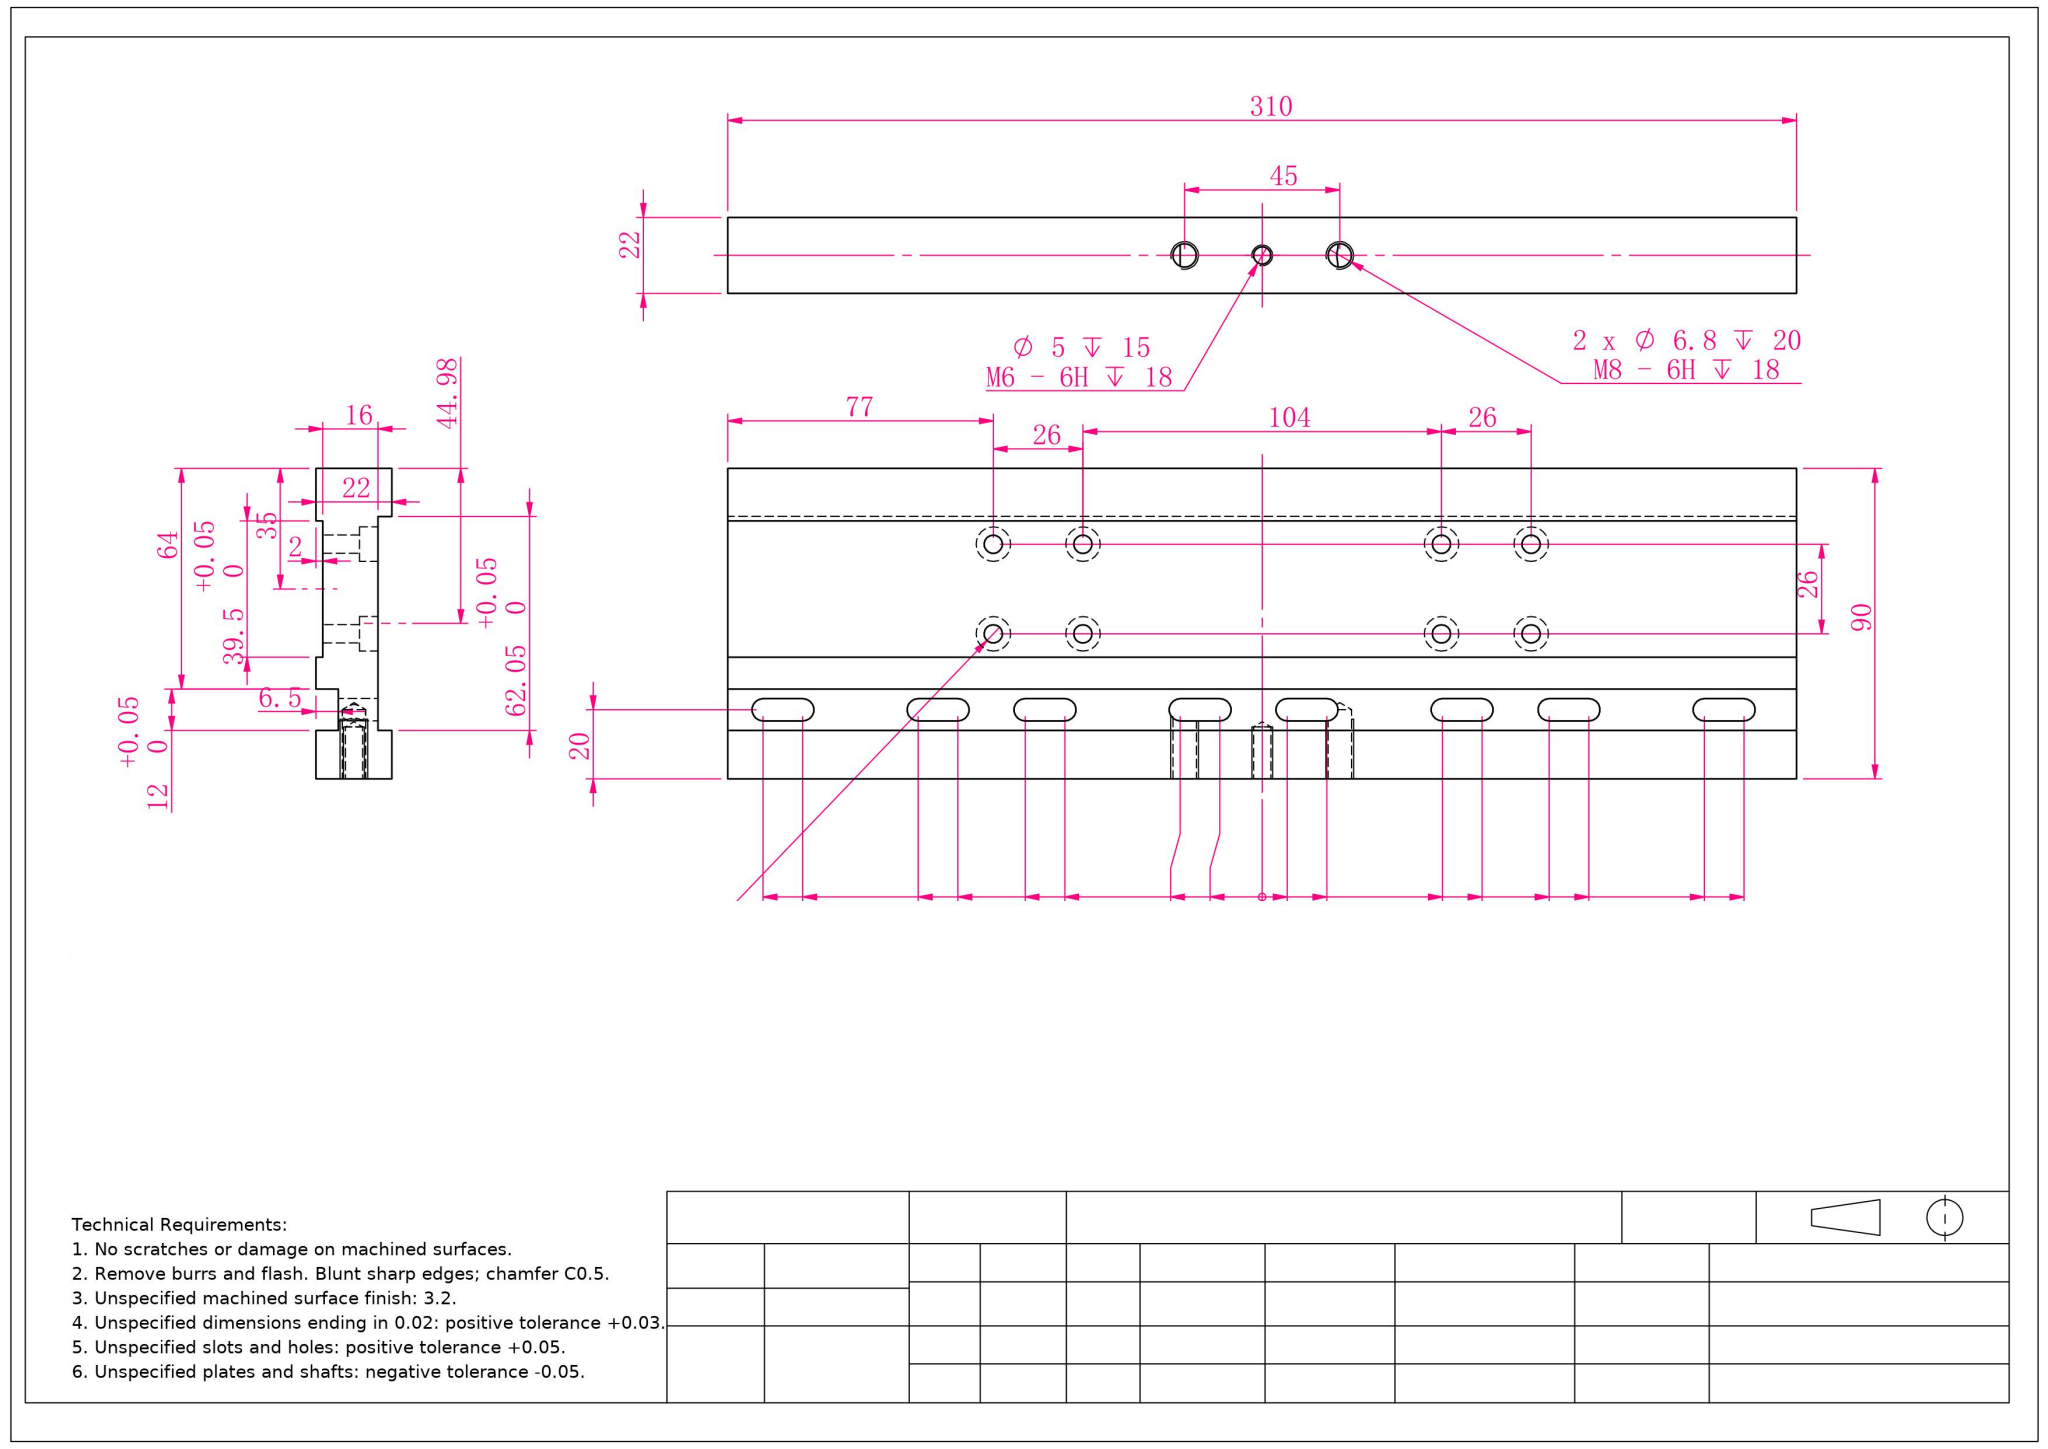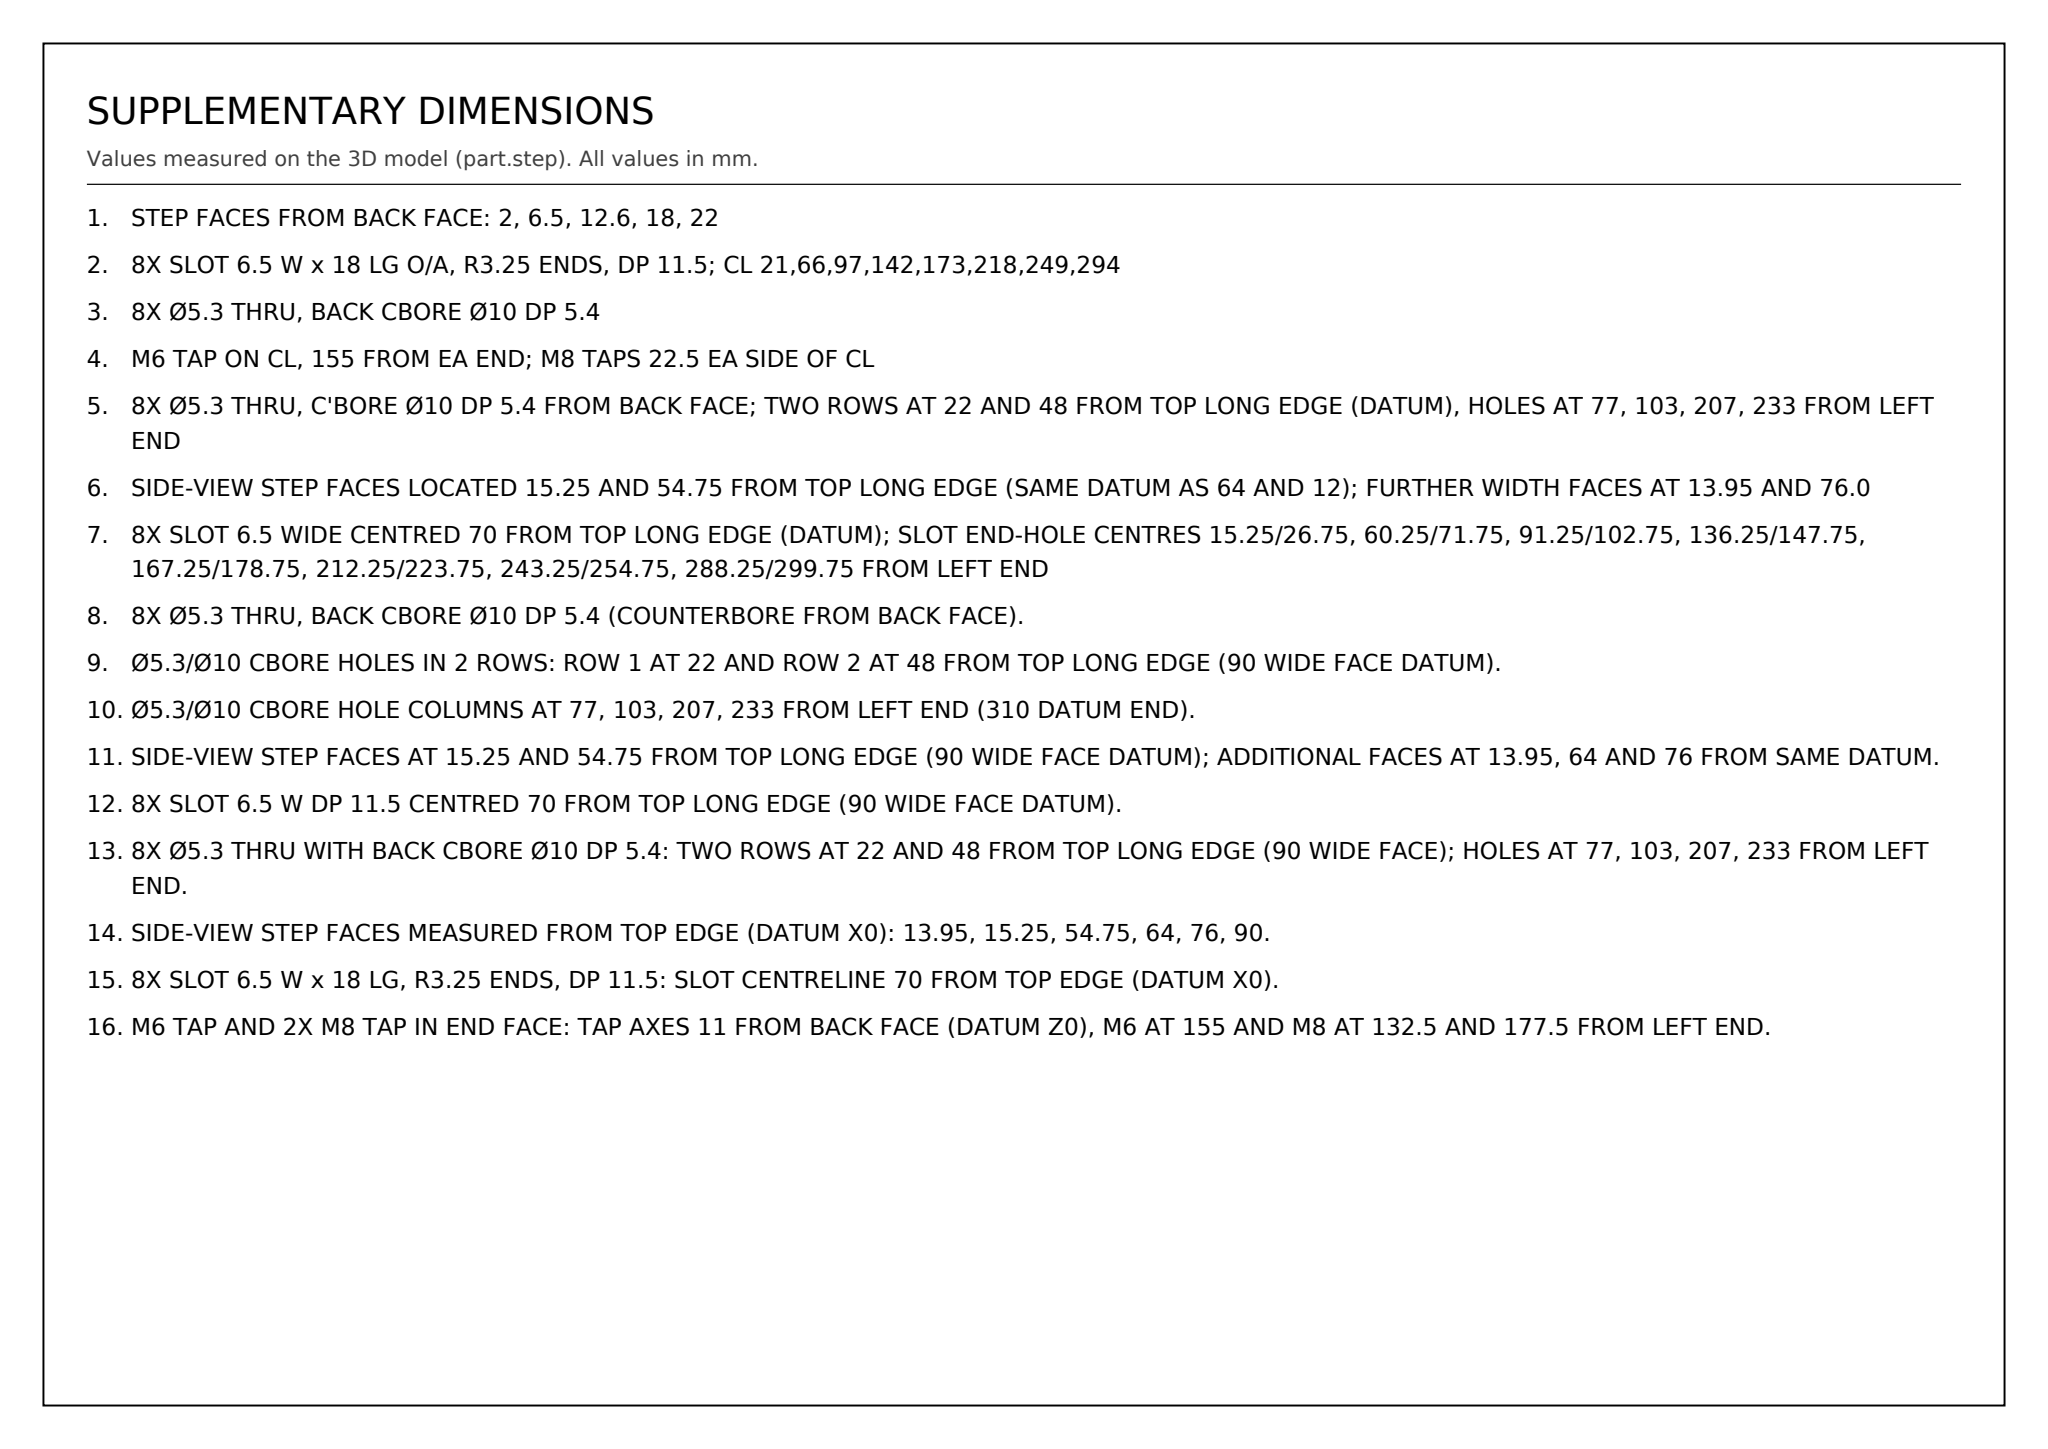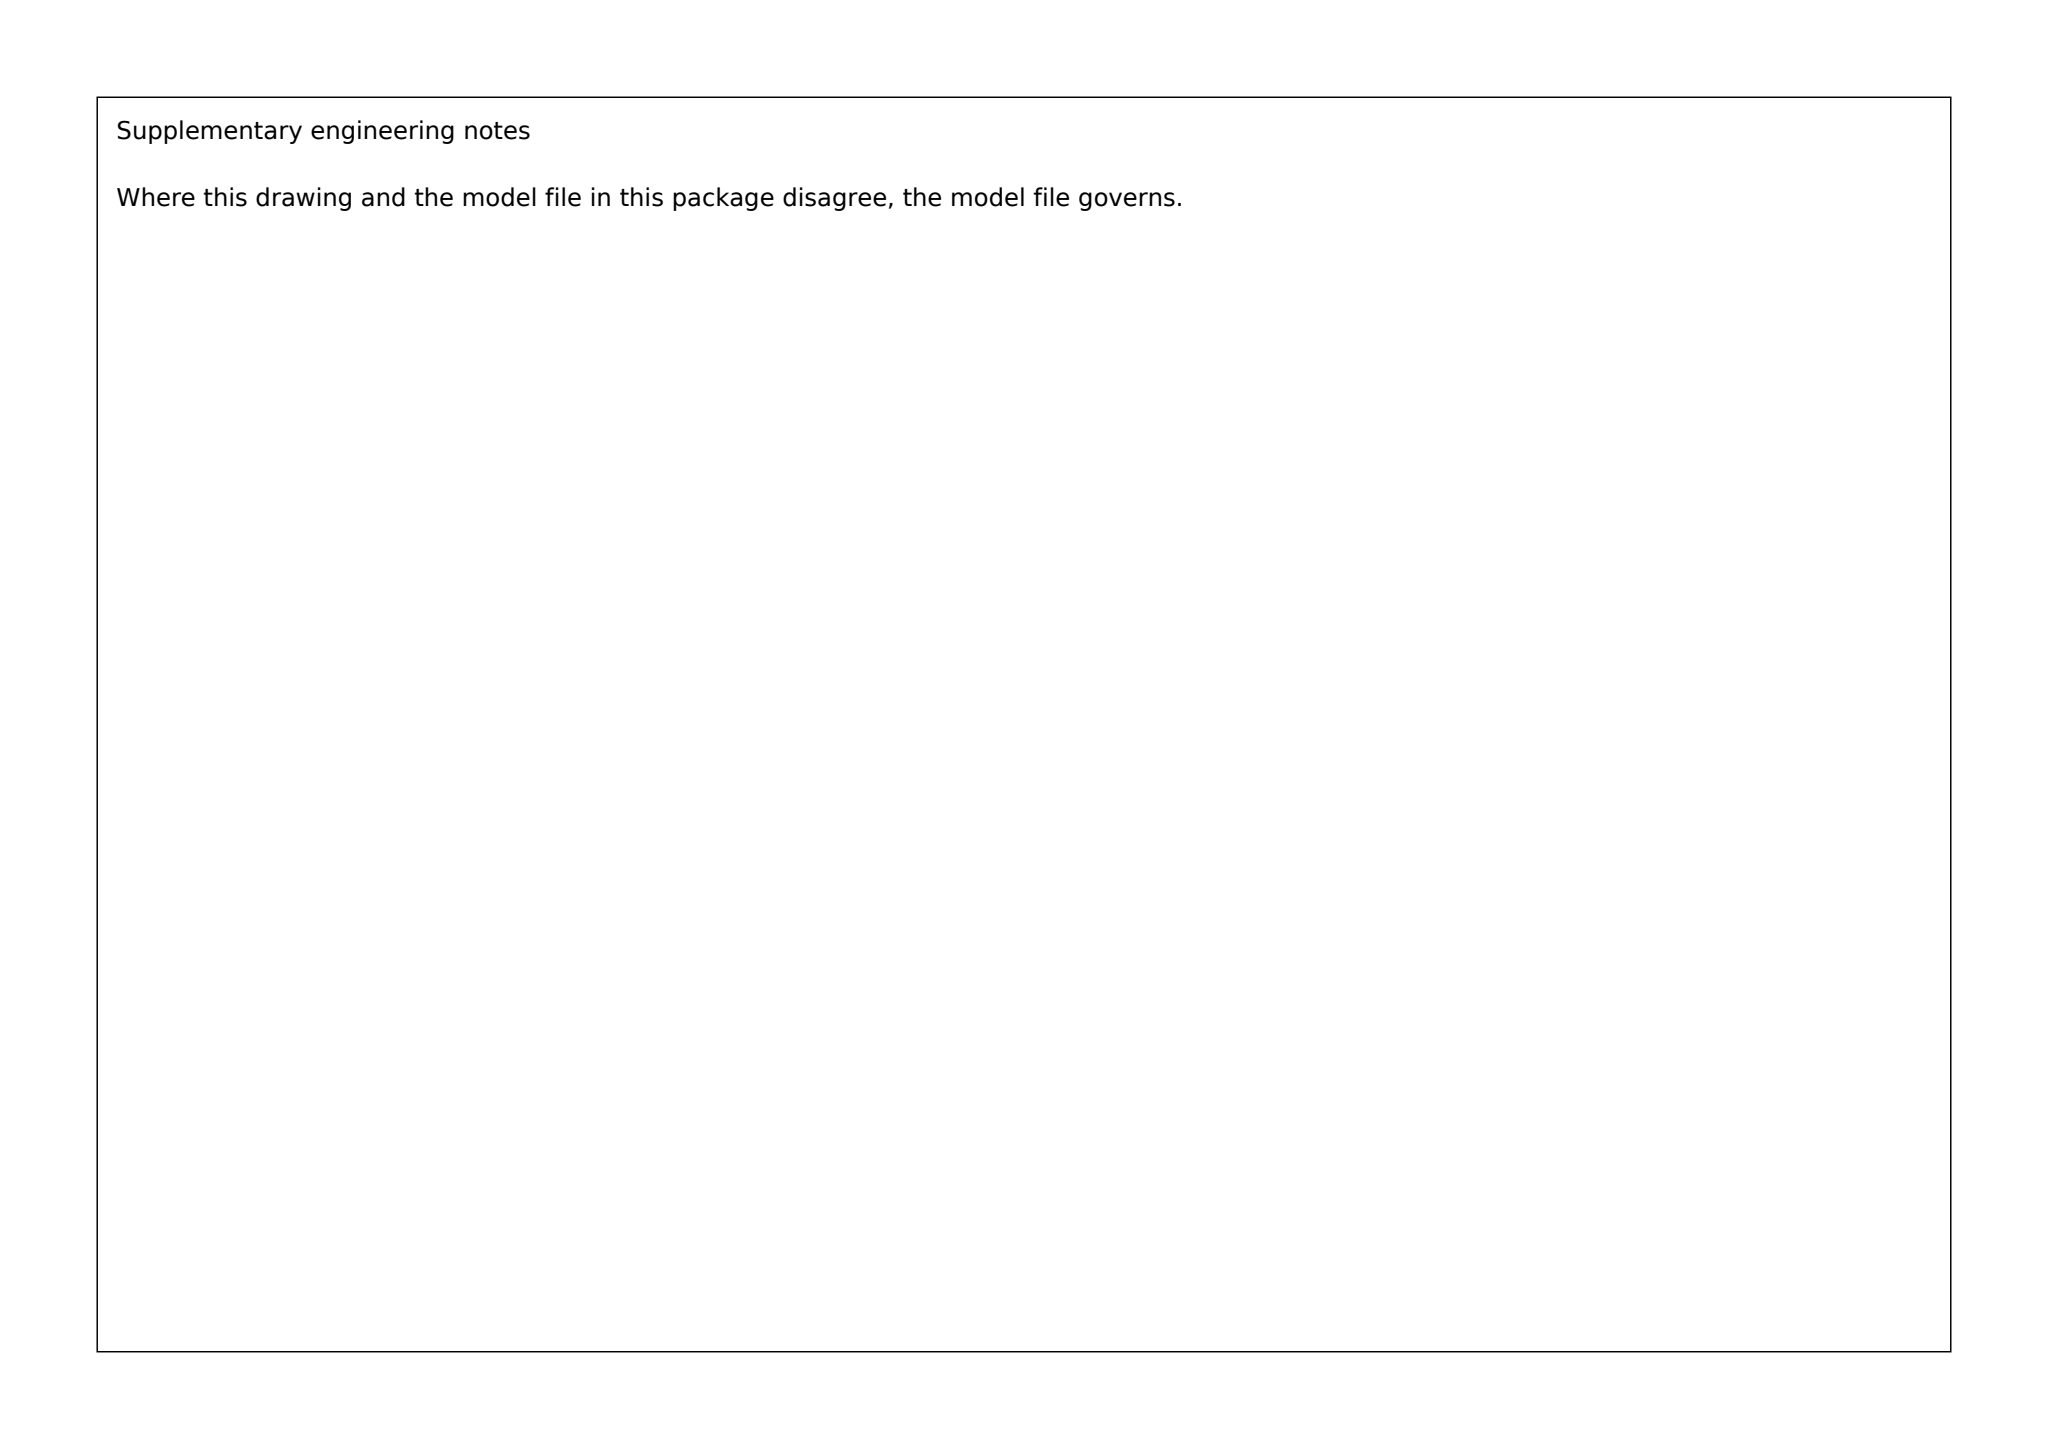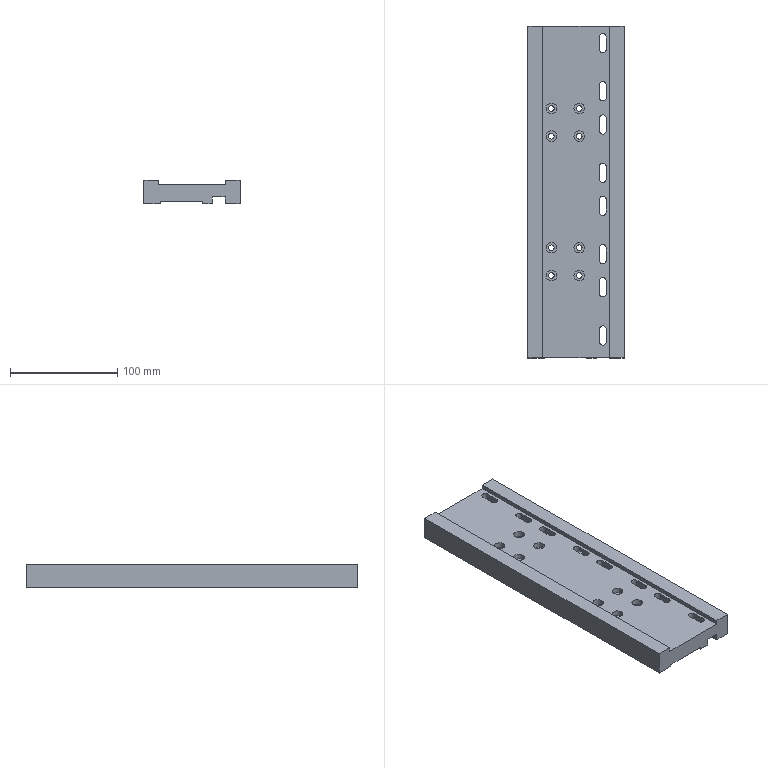Part | SolidWorks | mm | 1 solid | 100 faces | box 90 x 310 x 22 mm | volume 471371 mm3 | cylinder 54 | plane 42 | cone 4 | commonest cylinder face diameters 10 x16 5.3 x16 6.5 x16 6.8 x4 5 x2
Drawing notes:
STEP FACES FROM BACK FACE: 2, 6.5, 12.6, 18, 22 | from the solid: z-normal planes at 0, 2, 6.5, 12.6, 18, 22
8X SLOT 6.5 W x 18 LG O/A, R3.25 ENDS, DP 11.5; CL 21,66,97,142,173,218,249,294 | from the solid: Ø6.5 z-cyls at x=70, pairs 11.5 apart (y=15.25/26.75 ... 288.25/299.75), len 11.5; midpoints give CL
8X Ø5.3 THRU, BACK CBORE Ø10 DP 5.4 | from the solid: Ø5.3 z-cyls len 10.6 with Ø10 z-cyls len 5.4 at x=22/48, y=77/103/207/233
M6 TAP ON CL, 155 FROM EA END; M8 TAPS 22.5 EA SIDE OF CL | from the solid: Ø5 x-axis hole at y=155; Ø6.8 x-axis holes at y=132.5 & 177.5; bbox y=310
8X Ø5.3 THRU, C'BORE Ø10 DP 5.4 FROM BACK FACE; TWO ROWS AT 22 AND 48 FROM TOP LONG EDGE (DATUM), HOLES AT 77, 103, 207, 233 FROM LEFT END | from the solid: cylinders dia 5.3 z at (22,77),(22,103),(22,207),(22,233),(48,77),(48,103),(48,207),(48,233) L10.6 and dia 10.0 z same positions L5.4
SIDE-VIEW STEP FACES LOCATED 15.25 AND 54.75 FROM TOP LONG EDGE (SAME DATUM AS 64 AND 12); FURTHER WIDTH FACES AT 13.95 AND 76.0 | from the solid: axis_planes normal x at offsets 13.95, 15.25, 54.75, 76.0 (bbox x 0-90)
8X SLOT 6.5 WIDE CENTRED 70 FROM TOP LONG EDGE (DATUM); SLOT END-HOLE CENTRES 15.25/26.75, 60.25/71.75, 91.25/102.75, 136.25/147.75, 167.25/178.75, 212.25/223.75, 243.25/254.75, 288.25/299.75 FROM LEFT END | from the solid: cylinders dia 6.5 axis z at x=70.0, y=15.25...299.75, length 11.5
8X Ø5.3 THRU, BACK CBORE Ø10 DP 5.4 (COUNTERBORE FROM BACK FACE). | from the solid: cylinders dia 5.3 axis z length 10.6 (8 places) with coaxial dia 10.0 axis z length 5.4
Ø5.3/Ø10 CBORE HOLES IN 2 ROWS: ROW 1 AT 22 AND ROW 2 AT 48 FROM TOP LONG EDGE (90 WIDE FACE DATUM). | from the solid: cylinders dia 5.3 axis z pos_other_axes x = 22.0 and x = 48.0
Ø5.3/Ø10 CBORE HOLE COLUMNS AT 77, 103, 207, 233 FROM LEFT END (310 DATUM END). | from the solid: cylinders dia 5.3 axis z pos_other_axes y = 77.0, 103.0, 207.0, 233.0
SIDE-VIEW STEP FACES AT 15.25 AND 54.75 FROM TOP LONG EDGE (90 WIDE FACE DATUM); ADDITIONAL FACES AT 13.95, 64 AND 76 FROM SAME DATUM. | from the solid: axis_planes normal x at offsets 13.95, 15.25, 54.75, 64.0, 76.0 (edges at x = 0 and 90)
8X SLOT 6.5 W DP 11.5 CENTRED 70 FROM TOP LONG EDGE (90 WIDE FACE DATUM). | from the solid: cylinders dia 6.5 axis z pos_other_axes x = 70.0, length 11.5
8X Ø5.3 THRU WITH BACK CBORE Ø10 DP 5.4: TWO ROWS AT 22 AND 48 FROM TOP LONG EDGE (90 WIDE FACE); HOLES AT 77, 103, 207, 233 FROM LEFT END. | from the solid: cylinders Ø5.3 z-axis at (22,77),(22,103),(22,207),(22,233),(48,77),(48,103),(48,207),(48,233) and Ø10 z-axis DP 5.4 at same positions
SIDE-VIEW STEP FACES MEASURED FROM TOP EDGE (DATUM X0): 13.95, 15.25, 54.75, 64, 76, 90. | from the solid: axis_planes normal x at offsets 0, 13.95, 15.25, 54.75, 64, 76, 90
8X SLOT 6.5 W x 18 LG, R3.25 ENDS, DP 11.5: SLOT CENTRELINE 70 FROM TOP EDGE (DATUM X0). | from the solid: cylinders Ø6.5 z-axis all at x = 70.0, length 11.5
M6 TAP AND 2X M8 TAP IN END FACE: TAP AXES 11 FROM BACK FACE (DATUM Z0), M6 AT 155 AND M8 AT 132.5 AND 177.5 FROM LEFT END. | from the solid: cylinders Ø5.0 x-axis at (155,11) and Ø6.8 x-axis at (132.5,11) and (177.5,11)